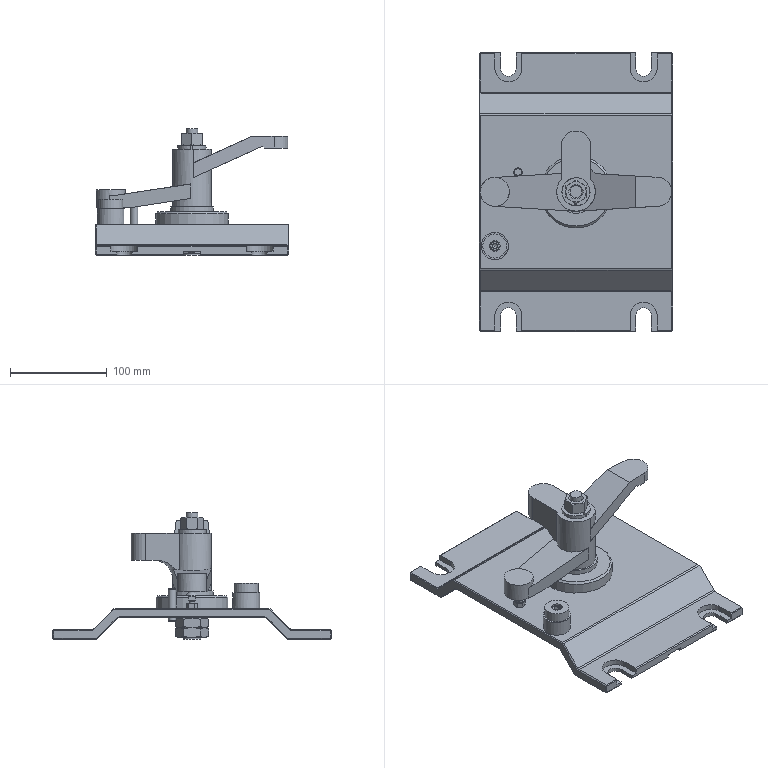Assembly | NX | mm | 10 component files | 12 solids | 327 faces | box 200 x 288 x 131 mm | volume 869279 mm3 | plane 205 | cone 72 | cylinder 46 | torus 3 | sphere 1 | commonest cylinder face diameters 16 x5 28 x5 20 x4 1 x4 30 x3 8 x3 6 x3 17.97 x3
Bill of materials:
GB12-88,M6x16 | 1 |  | Cup Head Square Neck Bolt, GB 12-88,M6x16
unnamed part 1 | 1 |  | Three-armed lever or crank-like part. It has a central cylindrical hub with a through bore. Two long tapered arms run out in opposite directions and end in rounded pads, and a shorter straight arm with a rounded end sticks out sideways from the hub. The arms sit at different heights.
GB-T6172_1-2000,M20x2.5 | 2 |  | Hexagon Thin Nut, Chamfered, GB-T 6172.1-2000,M20x2.5
GB-T6170_F-2000,M6x1 | 1 |  | Hexagonal prism with a central through bore and chamfered top and bottom edges. It is visibly flatter in proportion than unnamed part. Its shape is consistent with a hex nut.
GB-T70.1-2000,M6x12 | 1 |  | Hexagon Socket Head Cap Screw, GB-T 70.1-2000,M6x12
unnamed part 2 | 1 |  | Rectangular formed plate. Its middle section is raised, joggled up from lower flanges at two opposite ends, and each end flange has two open U-slots. On the raised section sit a stepped cylindrical shaft rising from a stepped circular boss, a smaller cylindrical boss with a hole, and a few small holes. Overall it is consistent with a base plate carrying a shaft, possibly a motor- or gearbox-like unit.
GB859-87,(18) | 1 |  | Single Coil spring Lock Washer, Light Type, GB 859-87,(18)
GB-T6170_F-2000,M14x2 | 1 |  | Hexagonal prism with a central through bore and chamfered end edges. It is proportionally taller than unnamed part. Its shape is consistent with a hex nut.
GB-T119.1-2000,8x35 | 1 |  | Parallel Pin, GB-T 119.1-2000,8x35
Mates:
1. touch align | GB-T6170_F-2000_M14x2 1 face | GB859-87__18 1 face
2. touch align | GB-T70_1-2000_M6x12 1 face | assembly face
3. touch align | GB-T70_1-2000_M6x12 1 face | assembly face
4. touch align | equal_arm_lever_blank 1 face | assembly face
5. touch align | equal_arm_lever_blank 1 face | assembly face
6. touch align | equal_arm_lever_blank 1 face | GB859-87__18 1 face
7. touch align | assembly face | GB-T6172_1-2000_M20x2_5 2 face
8. touch align | GB-T6170_F-2000_M6x1 1 face | GB12-88_M6x16 1 face
9. touch align | GB-T6170_F-2000_M6x1 1 face | assembly face